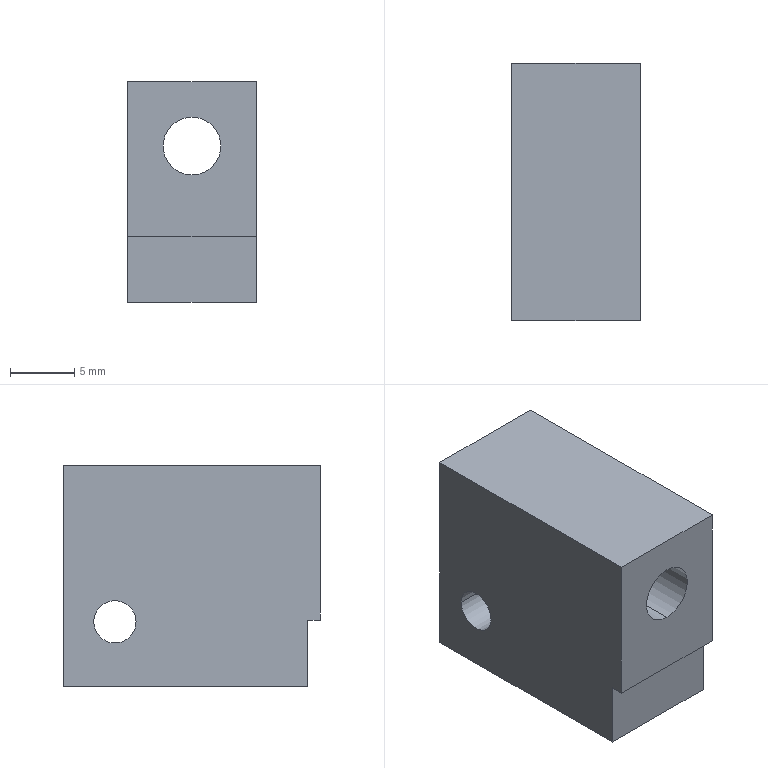Component | SolidWorks | 17268065-1 | 1 solid | 15 faces | box 10 x 20 x 17.15 mm | volume 2824 mm3 | plane 9 | cylinder 6 | commonest cylinder face diameters 3.3 x2 8 x2 4.5 x2 | material SKD-11 HRC58° Hard Chrome Plated
build123d program:
from build123d import *

# Parameters (mm, degrees)
SKETCH1_W                                       = 17.149
SKETCH1_H                                       = 10
BOSS_EXTRUDE1_DEPTH                             = 20
SKETCH2_W                                       = 5.149
SKETCH2_H                                       = 1
CUT_EXTRUDE1_DEPTH                              = 26.377
M4_HEX_SOCKET_HEAD_CAP_SCREW_CBORE1_D           = 4.5
M4_HEX_SOCKET_HEAD_CAP_SCREW_CBORE1_CBORE_D     = 8
M4_HEX_SOCKET_HEAD_CAP_SCREW_CBORE1_CBORE_DEPTH = 4.4
M4_TAPPED_HOLE1_D                               = 3.3


with BuildPart() as part:
    # Sketch1 → Boss-Extrude1 (new body)
    with BuildSketch(Plane.XY):
        with Locations((3.425, 108.5)):
            Rectangle(SKETCH1_W, SKETCH1_H)
    extrude(amount=BOSS_EXTRUDE1_DEPTH)

    # Sketch2 → Cut-Extrude1 (cut, through all)
    with BuildSketch(Plane(origin=(0, 113.5, 0), x_dir=(1, 0, 0), z_dir=(0, 1, 0))):
        with Locations((9.425, -0.5)):
            Rectangle(SKETCH2_W, SKETCH2_H)
    extrude(amount=-CUT_EXTRUDE1_DEPTH, mode=Mode.SUBTRACT)

    # M4 Hex Socket Head Cap Screw CBORE1 (through all)
    with Locations(Plane.XY.offset(20)):
        with Locations((-0.1493, 108.5)):
            CounterBoreHole(M4_HEX_SOCKET_HEAD_CAP_SCREW_CBORE1_D / 2, M4_HEX_SOCKET_HEAD_CAP_SCREW_CBORE1_CBORE_D / 2, M4_HEX_SOCKET_HEAD_CAP_SCREW_CBORE1_CBORE_DEPTH)

    # M4 Tapped Hole1 (through all)
    with Locations(Plane(origin=(0, 113.5, 0), x_dir=(1, 0, 0), z_dir=(0, 1, 0))):
        with Locations((7, -16)):
            Hole(M4_TAPPED_HOLE1_D / 2)


solid = part.part

# Placed as in the assembly
solid = solid.moved(Location((39.5, -43.579, 0.8507), (-90, 0, 90)))
STEP:
#1=COLOUR_RGB('',0.7922,0.8196,0.9333);
#2=FILL_AREA_STYLE_COLOUR('',#1);
#3=FILL_AREA_STYLE('',(#2));
#4=SURFACE_STYLE_FILL_AREA(#3);
#5=SURFACE_SIDE_STYLE('',(#4));
#6=SURFACE_STYLE_USAGE(.BOTH.,#5);
#7=PRESENTATION_STYLE_ASSIGNMENT((#6));
#8=CARTESIAN_POINT('',(-2.52,-1.151,-0.2421));
#9=VERTEX_POINT('',#8);
#10=CARTESIAN_POINT('',(-2.52,-1.021,-0.2421));
#11=VERTEX_POINT('',#10);
#12=CARTESIAN_POINT('',(-2.52,-1.086,-0.2421));
#13=DIRECTION('',(-1.,0.,0.));
#14=DIRECTION('',(0.,1.,0.));
#15=AXIS2_PLACEMENT_3D('',#12,#13,#14);
#16=CIRCLE('',#15,0.06496);
#17=EDGE_CURVE('',#9,#11,#16,.T.);
#18=ORIENTED_EDGE('',*,*,#17,.F.);
#19=CARTESIAN_POINT('',(-2.913,-1.151,-0.2421));
#20=VERTEX_POINT('',#19);
#21=CARTESIAN_POINT('',(-2.913,-1.151,-0.2421));
#22=DIRECTION('',(-1.,0.,0.));
#23=VECTOR('',#22,39.37);
#24=LINE('',#21,#23);
#25=EDGE_CURVE('',#9,#20,#24,.T.);
#26=ORIENTED_EDGE('',*,*,#25,.T.);
#27=CARTESIAN_POINT('',(-2.913,-1.021,-0.2421));
#28=VERTEX_POINT('',#27);
#29=CARTESIAN_POINT('',(-2.913,-1.086,-0.2421));
#30=DIRECTION('',(-1.,0.,0.));
#31=DIRECTION('',(0.,1.,0.));
#32=AXIS2_PLACEMENT_3D('',#29,#30,#31);
#33=CIRCLE('',#32,0.06496);
#34=EDGE_CURVE('',#20,#28,#33,.T.);
#35=ORIENTED_EDGE('',*,*,#34,.T.);
#36=CARTESIAN_POINT('',(-2.913,-1.021,-0.2421));
#37=DIRECTION('',(-1.,0.,0.));
#38=VECTOR('',#37,39.37);
#39=LINE('',#36,#38);
#40=EDGE_CURVE('',#11,#28,#39,.T.);
#41=ORIENTED_EDGE('',*,*,#40,.F.);
#42=EDGE_LOOP('',(#18,#26,#35,#41));
#43=FACE_OUTER_BOUND('',#42,.T.);
#44=CARTESIAN_POINT('',(-2.913,-1.086,-0.2421));
#45=DIRECTION('',(-1.,0.,0.));
#46=DIRECTION('',(0.,1.,0.));
#47=AXIS2_PLACEMENT_3D('',#44,#45,#46);
#48=CYLINDRICAL_SURFACE('',#47,0.06496);
#49=ADVANCED_FACE('',(#43),#48,.F.);
#50=CARTESIAN_POINT('',(-2.717,-1.102,0.1969));
#51=VERTEX_POINT('',#50);
#52=CARTESIAN_POINT('',(-2.717,-1.102,-0.1181));
#53=VERTEX_POINT('',#52);
#54=CARTESIAN_POINT('',(-2.717,-1.102,0.03937));
#55=DIRECTION('',(0.,1.,-0.));
#56=DIRECTION('',(0.,0.,-1.));
#57=AXIS2_PLACEMENT_3D('',#54,#55,#56);
#58=CIRCLE('',#57,0.1575);
#59=EDGE_CURVE('',#51,#53,#58,.T.);
#60=ORIENTED_EDGE('',*,*,#59,.F.);
#61=CARTESIAN_POINT('',(-2.717,-0.9283,0.1969));
#62=VERTEX_POINT('',#61);
#63=CARTESIAN_POINT('',(-2.717,-0.9283,0.1969));
#64=DIRECTION('',(0.,1.,-0.));
#65=VECTOR('',#64,39.37);
#66=LINE('',#63,#65);
#67=EDGE_CURVE('',#51,#62,#66,.T.);
#68=ORIENTED_EDGE('',*,*,#67,.T.);
#69=CARTESIAN_POINT('',(-2.717,-0.9283,-0.1181));
#70=VERTEX_POINT('',#69);
#71=CARTESIAN_POINT('',(-2.717,-0.9283,0.03937));
#72=DIRECTION('',(0.,1.,-0.));
#73=DIRECTION('',(0.,0.,-1.));
#74=AXIS2_PLACEMENT_3D('',#71,#72,#73);
#75=CIRCLE('',#74,0.1575);
#76=EDGE_CURVE('',#62,#70,#75,.T.);
#77=ORIENTED_EDGE('',*,*,#76,.T.);
#78=CARTESIAN_POINT('',(-2.717,-0.9283,-0.1181));
#79=DIRECTION('',(0.,1.,-0.));
#80=VECTOR('',#79,39.37);
#81=LINE('',#78,#80);
#82=EDGE_CURVE('',#53,#70,#81,.T.);
#83=ORIENTED_EDGE('',*,*,#82,.F.);
#84=EDGE_LOOP('',(#60,#68,#77,#83));
#85=FACE_OUTER_BOUND('',#84,.T.);
#86=CARTESIAN_POINT('',(-2.717,-0.9283,0.03937));
#87=DIRECTION('',(0.,1.,-0.));
#88=DIRECTION('',(0.,0.,-1.));
#89=AXIS2_PLACEMENT_3D('',#86,#87,#88);
#90=CYLINDRICAL_SURFACE('',#89,0.1575);
#91=ADVANCED_FACE('',(#85),#90,.F.);
#92=CARTESIAN_POINT('',(-2.717,-1.716,0.128));
#93=VERTEX_POINT('',#92);
#94=CARTESIAN_POINT('',(-2.717,-1.716,-0.04921));
#95=VERTEX_POINT('',#94);
#96=CARTESIAN_POINT('',(-2.717,-1.716,0.03937));
#97=DIRECTION('',(0.,1.,-0.));
#98=DIRECTION('',(0.,0.,-1.));
#99=AXIS2_PLACEMENT_3D('',#96,#97,#98);
#100=CIRCLE('',#99,0.08858);
#101=EDGE_CURVE('',#93,#95,#100,.T.);
#102=ORIENTED_EDGE('',*,*,#101,.F.);
#103=CARTESIAN_POINT('',(-2.717,-1.102,0.128));
#104=VERTEX_POINT('',#103);
#105=CARTESIAN_POINT('',(-2.717,-0.9283,0.128));
#106=DIRECTION('',(0.,1.,-0.));
#107=VECTOR('',#106,39.37);
#108=LINE('',#105,#107);
#109=EDGE_CURVE('',#93,#104,#108,.T.);
#110=ORIENTED_EDGE('',*,*,#109,.T.);
#111=CARTESIAN_POINT('',(-2.717,-1.102,-0.04921));
#112=VERTEX_POINT('',#111);
#113=CARTESIAN_POINT('',(-2.717,-1.102,0.03937));
#114=DIRECTION('',(0.,1.,-0.));
#115=DIRECTION('',(0.,0.,-1.));
#116=AXIS2_PLACEMENT_3D('',#113,#114,#115);
#117=CIRCLE('',#116,0.08858);
#118=EDGE_CURVE('',#104,#112,#117,.T.);
#119=ORIENTED_EDGE('',*,*,#118,.T.);
#120=CARTESIAN_POINT('',(-2.717,-0.9283,-0.04921));
#121=DIRECTION('',(0.,1.,-0.));
#122=VECTOR('',#121,39.37);
#123=LINE('',#120,#122);
#124=EDGE_CURVE('',#95,#112,#123,.T.);
#125=ORIENTED_EDGE('',*,*,#124,.F.);
#126=EDGE_LOOP('',(#102,#110,#119,#125));
#127=FACE_OUTER_BOUND('',#126,.T.);
#128=CARTESIAN_POINT('',(-2.717,-0.9283,0.03937));
#129=DIRECTION('',(0.,1.,-0.));
#130=DIRECTION('',(0.,0.,-1.));
#131=AXIS2_PLACEMENT_3D('',#128,#129,#130);
#132=CYLINDRICAL_SURFACE('',#131,0.08858);
#133=ADVANCED_FACE('',(#127),#132,.F.);
#134=CARTESIAN_POINT('',(-2.913,-1.716,0.2362));
#135=VERTEX_POINT('',#134);
#136=CARTESIAN_POINT('',(-2.52,-1.716,0.2362));
#137=VERTEX_POINT('',#136);
#138=CARTESIAN_POINT('',(-2.913,-1.716,0.2362));
#139=DIRECTION('',(1.,-0.,-0.));
#140=VECTOR('',#139,39.37);
#141=LINE('',#138,#140);
#142=EDGE_CURVE('',#135,#137,#141,.T.);
#143=ORIENTED_EDGE('',*,*,#142,.T.);
#144=CARTESIAN_POINT('',(-2.52,-0.9283,0.2362));
#145=VERTEX_POINT('',#144);
#146=CARTESIAN_POINT('',(-2.52,-0.9283,0.2362));
#147=DIRECTION('',(0.,-1.,0.));
#148=VECTOR('',#147,39.37);
#149=LINE('',#146,#148);
#150=EDGE_CURVE('',#145,#137,#149,.T.);
#151=ORIENTED_EDGE('',*,*,#150,.F.);
#152=CARTESIAN_POINT('',(-2.913,-0.9283,0.2362));
#153=VERTEX_POINT('',#152);
#154=CARTESIAN_POINT('',(-2.913,-0.9283,0.2362));
#155=DIRECTION('',(1.,-0.,-0.));
#156=VECTOR('',#155,39.37);
#157=LINE('',#154,#156);
#158=EDGE_CURVE('',#153,#145,#157,.T.);
#159=ORIENTED_EDGE('',*,*,#158,.F.);
#160=CARTESIAN_POINT('',(-2.913,-0.9283,0.2362));
#161=DIRECTION('',(0.,-1.,0.));
#162=VECTOR('',#161,39.37);
#163=LINE('',#160,#162);
#164=EDGE_CURVE('',#153,#135,#163,.T.);
#165=ORIENTED_EDGE('',*,*,#164,.T.);
#166=EDGE_LOOP('',(#143,#151,#159,#165));
#167=FACE_OUTER_BOUND('',#166,.T.);
#168=CARTESIAN_POINT('',(-2.913,-0.9283,0.2362));
#169=DIRECTION('',(-0.,-0.,-1.));
#170=DIRECTION('',(-1.,0.,0.));
#171=AXIS2_PLACEMENT_3D('',#168,#169,#170);
#172=PLANE('',#171);
#173=ADVANCED_FACE('',(#167),#172,.F.);
#174=CARTESIAN_POINT('',(-2.52,-1.086,-0.2421));
#175=DIRECTION('',(-1.,0.,0.));
#176=DIRECTION('',(0.,1.,0.));
#177=AXIS2_PLACEMENT_3D('',#174,#175,#176);
#178=CIRCLE('',#177,0.06496);
#179=EDGE_CURVE('',#11,#9,#178,.T.);
#180=ORIENTED_EDGE('',*,*,#179,.T.);
#181=ORIENTED_EDGE('',*,*,#17,.T.);
#182=EDGE_LOOP('',(#180,#181));
#183=FACE_BOUND('',#182,.T.);
#184=CARTESIAN_POINT('',(-2.52,-1.716,-0.2362));
#185=VERTEX_POINT('',#184);
#186=CARTESIAN_POINT('',(-2.52,-1.716,0.2362));
#187=DIRECTION('',(0.,-0.,-1.));
#188=VECTOR('',#187,39.37);
#189=LINE('',#186,#188);
#190=EDGE_CURVE('',#137,#185,#189,.T.);
#191=ORIENTED_EDGE('',*,*,#190,.T.);
#192=CARTESIAN_POINT('',(-2.52,-1.676,-0.2362));
#193=VERTEX_POINT('',#192);
#194=CARTESIAN_POINT('',(-2.52,-1.716,-0.2362));
#195=DIRECTION('',(0.,1.,-0.));
#196=VECTOR('',#195,39.37);
#197=LINE('',#194,#196);
#198=EDGE_CURVE('',#185,#193,#197,.T.);
#199=ORIENTED_EDGE('',*,*,#198,.T.);
#200=CARTESIAN_POINT('',(-2.52,-1.676,-0.4389));
#201=VERTEX_POINT('',#200);
#202=CARTESIAN_POINT('',(-2.52,-1.676,-0.2362));
#203=DIRECTION('',(0.,-0.,-1.));
#204=VECTOR('',#203,39.37);
#205=LINE('',#202,#204);
#206=EDGE_CURVE('',#193,#201,#205,.T.);
#207=ORIENTED_EDGE('',*,*,#206,.T.);
#208=CARTESIAN_POINT('',(-2.52,-0.9283,-0.4389));
#209=VERTEX_POINT('',#208);
#210=CARTESIAN_POINT('',(-2.52,-0.9283,-0.4389));
#211=DIRECTION('',(0.,-1.,0.));
#212=VECTOR('',#211,39.37);
#213=LINE('',#210,#212);
#214=EDGE_CURVE('',#209,#201,#213,.T.);
#215=ORIENTED_EDGE('',*,*,#214,.F.);
#216=CARTESIAN_POINT('',(-2.52,-0.9283,0.2362));
#217=DIRECTION('',(0.,-0.,-1.));
#218=VECTOR('',#217,39.37);
#219=LINE('',#216,#218);
#220=EDGE_CURVE('',#145,#209,#219,.T.);
#221=ORIENTED_EDGE('',*,*,#220,.F.);
#222=ORIENTED_EDGE('',*,*,#150,.T.);
#223=EDGE_LOOP('',(#191,#199,#207,#215,#221,#222));
#224=FACE_OUTER_BOUND('',#223,.T.);
#225=CARTESIAN_POINT('',(-2.52,-0.9283,0.2362));
#226=DIRECTION('',(-1.,0.,0.));
#227=DIRECTION('',(0.,1.,-0.));
#228=AXIS2_PLACEMENT_3D('',#225,#226,#227);
#229=PLANE('',#228);
#230=ADVANCED_FACE('',(#183,#224),#229,.F.);
#231=ORIENTED_EDGE('',*,*,#214,.T.);
#232=CARTESIAN_POINT('',(-2.913,-1.676,-0.4389));
#233=VERTEX_POINT('',#232);
#234=CARTESIAN_POINT('',(-2.52,-1.676,-0.4389));
#235=DIRECTION('',(-1.,0.,0.));
#236=VECTOR('',#235,39.37);
#237=LINE('',#234,#236);
#238=EDGE_CURVE('',#201,#233,#237,.T.);
#239=ORIENTED_EDGE('',*,*,#238,.T.);
#240=CARTESIAN_POINT('',(-2.913,-0.9283,-0.4389));
#241=VERTEX_POINT('',#240);
#242=CARTESIAN_POINT('',(-2.913,-0.9283,-0.4389));
#243=DIRECTION('',(0.,-1.,0.));
#244=VECTOR('',#243,39.37);
#245=LINE('',#242,#244);
#246=EDGE_CURVE('',#241,#233,#245,.T.);
#247=ORIENTED_EDGE('',*,*,#246,.F.);
#248=CARTESIAN_POINT('',(-2.913,-0.9283,-0.4389));
#249=DIRECTION('',(-1.,0.,0.));
#250=VECTOR('',#249,39.37);
#251=LINE('',#248,#250);
#252=EDGE_CURVE('',#209,#241,#251,.T.);
#253=ORIENTED_EDGE('',*,*,#252,.F.);
#254=EDGE_LOOP('',(#231,#239,#247,#253));
#255=FACE_OUTER_BOUND('',#254,.T.);
#256=CARTESIAN_POINT('',(-2.913,-0.9283,-0.4389));
#257=DIRECTION('',(0.,0.,1.));
#258=DIRECTION('',(0.,1.,-0.));
#259=AXIS2_PLACEMENT_3D('',#256,#257,#258);
#260=PLANE('',#259);
#261=ADVANCED_FACE('',(#255),#260,.F.);
#262=CARTESIAN_POINT('',(-2.913,-1.086,-0.2421));
#263=DIRECTION('',(-1.,0.,0.));
#264=DIRECTION('',(0.,1.,0.));
#265=AXIS2_PLACEMENT_3D('',#262,#263,#264);
#266=CIRCLE('',#265,0.06496);
#267=EDGE_CURVE('',#28,#20,#266,.T.);
#268=ORIENTED_EDGE('',*,*,#267,.F.);
#269=ORIENTED_EDGE('',*,*,#34,.F.);
#270=EDGE_LOOP('',(#268,#269));
#271=FACE_BOUND('',#270,.T.);
#272=CARTESIAN_POINT('',(-2.913,-1.676,-0.2362));
#273=VERTEX_POINT('',#272);
#274=CARTESIAN_POINT('',(-2.913,-1.676,-0.2362));
#275=DIRECTION('',(0.,-0.,-1.));
#276=VECTOR('',#275,39.37);
#277=LINE('',#274,#276);
#278=EDGE_CURVE('',#273,#233,#277,.T.);
#279=ORIENTED_EDGE('',*,*,#278,.F.);
#280=CARTESIAN_POINT('',(-2.913,-1.716,-0.2362));
#281=VERTEX_POINT('',#280);
#282=CARTESIAN_POINT('',(-2.913,-1.716,-0.2362));
#283=DIRECTION('',(0.,1.,-0.));
#284=VECTOR('',#283,39.37);
#285=LINE('',#282,#284);
#286=EDGE_CURVE('',#281,#273,#285,.T.);
#287=ORIENTED_EDGE('',*,*,#286,.F.);
#288=CARTESIAN_POINT('',(-2.913,-1.716,0.2362));
#289=DIRECTION('',(0.,0.,1.));
#290=VECTOR('',#289,39.37);
#291=LINE('',#288,#290);
#292=EDGE_CURVE('',#281,#135,#291,.T.);
#293=ORIENTED_EDGE('',*,*,#292,.T.);
#294=ORIENTED_EDGE('',*,*,#164,.F.);
#295=CARTESIAN_POINT('',(-2.913,-0.9283,0.2362));
#296=DIRECTION('',(0.,0.,1.));
#297=VECTOR('',#296,39.37);
#298=LINE('',#295,#297);
#299=EDGE_CURVE('',#241,#153,#298,.T.);
#300=ORIENTED_EDGE('',*,*,#299,.F.);
#301=ORIENTED_EDGE('',*,*,#246,.T.);
#302=EDGE_LOOP('',(#279,#287,#293,#294,#300,#301));
#303=FACE_OUTER_BOUND('',#302,.T.);
#304=CARTESIAN_POINT('',(-2.913,-0.9283,0.2362));
#305=DIRECTION('',(1.,0.,0.));
#306=DIRECTION('',(0.,-1.,0.));
#307=AXIS2_PLACEMENT_3D('',#304,#305,#306);
#308=PLANE('',#307);
#309=ADVANCED_FACE('',(#271,#303),#308,.F.);
#310=CARTESIAN_POINT('',(-2.717,-0.9283,0.03937));
#311=DIRECTION('',(0.,1.,-0.));
#312=DIRECTION('',(0.,0.,-1.));
#313=AXIS2_PLACEMENT_3D('',#310,#311,#312);
#314=CIRCLE('',#313,0.1575);
#315=EDGE_CURVE('',#70,#62,#314,.T.);
#316=ORIENTED_EDGE('',*,*,#315,.F.);
#317=ORIENTED_EDGE('',*,*,#76,.F.);
#318=EDGE_LOOP('',(#316,#317));
#319=FACE_BOUND('',#318,.T.);
#320=ORIENTED_EDGE('',*,*,#158,.T.);
#321=ORIENTED_EDGE('',*,*,#220,.T.);
#322=ORIENTED_EDGE('',*,*,#252,.T.);
#323=ORIENTED_EDGE('',*,*,#299,.T.);
#324=EDGE_LOOP('',(#320,#321,#322,#323));
#325=FACE_OUTER_BOUND('',#324,.T.);
#326=CARTESIAN_POINT('',(1.555,-0.9283,0.03349));
#327=DIRECTION('',(0.,1.,-0.));
#328=DIRECTION('',(0.,-0.,-1.));
#329=AXIS2_PLACEMENT_3D('',#326,#327,#328);
#330=PLANE('',#329);
#331=ADVANCED_FACE('',(#319,#325),#330,.T.);
#332=CARTESIAN_POINT('',(-2.717,-1.716,0.03937));
#333=DIRECTION('',(0.,1.,-0.));
#334=DIRECTION('',(0.,0.,-1.));
#335=AXIS2_PLACEMENT_3D('',#332,#333,#334);
#336=CIRCLE('',#335,0.08858);
#337=EDGE_CURVE('',#95,#93,#336,.T.);
#338=ORIENTED_EDGE('',*,*,#337,.T.);
#339=ORIENTED_EDGE('',*,*,#101,.T.);
#340=EDGE_LOOP('',(#338,#339));
#341=FACE_BOUND('',#340,.T.);
#342=ORIENTED_EDGE('',*,*,#292,.F.);
#343=CARTESIAN_POINT('',(-2.52,-1.716,-0.2362));
#344=DIRECTION('',(-1.,0.,0.));
#345=VECTOR('',#344,39.37);
#346=LINE('',#343,#345);
#347=EDGE_CURVE('',#185,#281,#346,.T.);
#348=ORIENTED_EDGE('',*,*,#347,.F.);
#349=ORIENTED_EDGE('',*,*,#190,.F.);
#350=ORIENTED_EDGE('',*,*,#142,.F.);
#351=EDGE_LOOP('',(#342,#348,#349,#350));
#352=FACE_OUTER_BOUND('',#351,.T.);
#353=CARTESIAN_POINT('',(1.555,-1.716,0.03349));
#354=DIRECTION('',(0.,1.,-0.));
#355=DIRECTION('',(0.,-0.,-1.));
#356=AXIS2_PLACEMENT_3D('',#353,#354,#355);
#357=PLANE('',#356);
#358=ADVANCED_FACE('',(#341,#352),#357,.F.);
#359=ORIENTED_EDGE('',*,*,#286,.T.);
#360=CARTESIAN_POINT('',(-2.52,-1.676,-0.2362));
#361=DIRECTION('',(-1.,0.,0.));
#362=VECTOR('',#361,39.37);
#363=LINE('',#360,#362);
#364=EDGE_CURVE('',#193,#273,#363,.T.);
#365=ORIENTED_EDGE('',*,*,#364,.F.);
#366=ORIENTED_EDGE('',*,*,#198,.F.);
#367=ORIENTED_EDGE('',*,*,#347,.T.);
#368=EDGE_LOOP('',(#359,#365,#366,#367));
#369=FACE_OUTER_BOUND('',#368,.T.);
#370=CARTESIAN_POINT('',(-2.52,-1.716,-0.2362));
#371=DIRECTION('',(0.,0.,1.));
#372=DIRECTION('',(0.,1.,-0.));
#373=AXIS2_PLACEMENT_3D('',#370,#371,#372);
#374=PLANE('',#373);
#375=ADVANCED_FACE('',(#369),#374,.F.);
#376=ORIENTED_EDGE('',*,*,#278,.T.);
#377=ORIENTED_EDGE('',*,*,#238,.F.);
#378=ORIENTED_EDGE('',*,*,#206,.F.);
#379=ORIENTED_EDGE('',*,*,#364,.T.);
#380=EDGE_LOOP('',(#376,#377,#378,#379));
#381=FACE_OUTER_BOUND('',#380,.T.);
#382=CARTESIAN_POINT('',(-2.52,-1.676,-0.2362));
#383=DIRECTION('',(0.,1.,-0.));
#384=DIRECTION('',(0.,-0.,-1.));
#385=AXIS2_PLACEMENT_3D('',#382,#383,#384);
#386=PLANE('',#385);
#387=ADVANCED_FACE('',(#381),#386,.F.);
#388=ORIENTED_EDGE('',*,*,#109,.F.);
#389=ORIENTED_EDGE('',*,*,#337,.F.);
#390=ORIENTED_EDGE('',*,*,#124,.T.);
#391=CARTESIAN_POINT('',(-2.717,-1.102,0.03937));
#392=DIRECTION('',(0.,1.,-0.));
#393=DIRECTION('',(0.,0.,-1.));
#394=AXIS2_PLACEMENT_3D('',#391,#392,#393);
#395=CIRCLE('',#394,0.08858);
#396=EDGE_CURVE('',#112,#104,#395,.T.);
#397=ORIENTED_EDGE('',*,*,#396,.T.);
#398=EDGE_LOOP('',(#388,#389,#390,#397));
#399=FACE_OUTER_BOUND('',#398,.T.);
#400=CARTESIAN_POINT('',(-2.717,-0.9283,0.03937));
#401=DIRECTION('',(0.,1.,-0.));
#402=DIRECTION('',(0.,0.,-1.));
#403=AXIS2_PLACEMENT_3D('',#400,#401,#402);
#404=CYLINDRICAL_SURFACE('',#403,0.08858);
#405=ADVANCED_FACE('',(#399),#404,.F.);
#406=ORIENTED_EDGE('',*,*,#396,.F.);
#407=ORIENTED_EDGE('',*,*,#118,.F.);
#408=EDGE_LOOP('',(#406,#407));
#409=FACE_BOUND('',#408,.T.);
#410=CARTESIAN_POINT('',(-2.717,-1.102,0.03937));
#411=DIRECTION('',(0.,1.,-0.));
#412=DIRECTION('',(0.,0.,-1.));
#413=AXIS2_PLACEMENT_3D('',#410,#411,#412);
#414=CIRCLE('',#413,0.1575);
#415=EDGE_CURVE('',#53,#51,#414,.T.);
#416=ORIENTED_EDGE('',*,*,#415,.T.);
#417=ORIENTED_EDGE('',*,*,#59,.T.);
#418=EDGE_LOOP('',(#416,#417));
#419=FACE_OUTER_BOUND('',#418,.T.);
#420=CARTESIAN_POINT('',(-2.717,-1.102,-0.04921));
#421=DIRECTION('',(0.,-1.,0.));
#422=DIRECTION('',(0.,0.,1.));
#423=AXIS2_PLACEMENT_3D('',#420,#421,#422);
#424=PLANE('',#423);
#425=ADVANCED_FACE('',(#409,#419),#424,.F.);
#426=ORIENTED_EDGE('',*,*,#67,.F.);
#427=ORIENTED_EDGE('',*,*,#415,.F.);
#428=ORIENTED_EDGE('',*,*,#82,.T.);
#429=ORIENTED_EDGE('',*,*,#315,.T.);
#430=EDGE_LOOP('',(#426,#427,#428,#429));
#431=FACE_OUTER_BOUND('',#430,.T.);
#432=CARTESIAN_POINT('',(-2.717,-0.9283,0.03937));
#433=DIRECTION('',(0.,1.,-0.));
#434=DIRECTION('',(0.,0.,-1.));
#435=AXIS2_PLACEMENT_3D('',#432,#433,#434);
#436=CYLINDRICAL_SURFACE('',#435,0.1575);
#437=ADVANCED_FACE('',(#431),#436,.F.);
#438=ORIENTED_EDGE('',*,*,#25,.F.);
#439=ORIENTED_EDGE('',*,*,#179,.F.);
#440=ORIENTED_EDGE('',*,*,#40,.T.);
#441=ORIENTED_EDGE('',*,*,#267,.T.);
#442=EDGE_LOOP('',(#438,#439,#440,#441));
#443=FACE_OUTER_BOUND('',#442,.T.);
#444=CARTESIAN_POINT('',(-2.913,-1.086,-0.2421));
#445=DIRECTION('',(-1.,0.,0.));
#446=DIRECTION('',(0.,1.,0.));
#447=AXIS2_PLACEMENT_3D('',#444,#445,#446);
#448=CYLINDRICAL_SURFACE('',#447,0.06496);
#449=ADVANCED_FACE('',(#443),#448,.F.);
#450=CLOSED_SHELL('',(#49,#91,#133,#173,#230,#261,#309,#331,#358,#375,#387,#405,#425,#437,#449));
#451=MANIFOLD_SOLID_BREP('',#450);
#452=STYLED_ITEM('',(#7),#451);
#453=PRESENTATION_LAYER_ASSIGNMENT('','',(#452));
#454=(LENGTH_UNIT()NAMED_UNIT(*)SI_UNIT($,.METRE.));
#455=LENGTH_MEASURE_WITH_UNIT(LENGTH_MEASURE(0.0254),#454);
#456=DIMENSIONAL_EXPONENTS(1.,0.,0.,0.,0.,0.,0.);
#457=(CONVERSION_BASED_UNIT('',#455)LENGTH_UNIT()NAMED_UNIT(#456));
#458=UNCERTAINTY_MEASURE_WITH_UNIT(LENGTH_MEASURE(0.00001),#457,'','');
#459=(NAMED_UNIT(*)PLANE_ANGLE_UNIT()SI_UNIT($,.RADIAN.));
#460=(NAMED_UNIT(*)SI_UNIT($,.STERADIAN.)SOLID_ANGLE_UNIT());
#461=(GEOMETRIC_REPRESENTATION_CONTEXT(3)GLOBAL_UNCERTAINTY_ASSIGNED_CONTEXT((#458))GLOBAL_UNIT_ASSIGNED_CONTEXT((#457,#459,#460))REPRESENTATION_CONTEXT('',''));
#462=MECHANICAL_DESIGN_GEOMETRIC_PRESENTATION_REPRESENTATION('',(#452),#461);
#463=CARTESIAN_POINT('',(0.,0.,0.));
#464=DIRECTION('',(0.,0.,1.));
#465=DIRECTION('',(1.,0.,0.));
#466=AXIS2_PLACEMENT_3D('',#463,#464,#465);
#467=(LENGTH_UNIT()NAMED_UNIT(*)SI_UNIT($,.METRE.));
#468=LENGTH_MEASURE_WITH_UNIT(LENGTH_MEASURE(0.0254),#467);
#469=DIMENSIONAL_EXPONENTS(1.,0.,0.,0.,0.,0.,0.);
#470=(CONVERSION_BASED_UNIT('',#468)LENGTH_UNIT()NAMED_UNIT(#469));
#471=UNCERTAINTY_MEASURE_WITH_UNIT(LENGTH_MEASURE(0.00001),#470,'','');
#472=(NAMED_UNIT(*)PLANE_ANGLE_UNIT()SI_UNIT($,.RADIAN.));
#473=(NAMED_UNIT(*)SI_UNIT($,.STERADIAN.)SOLID_ANGLE_UNIT());
#474=(GEOMETRIC_REPRESENTATION_CONTEXT(3)GLOBAL_UNCERTAINTY_ASSIGNED_CONTEXT((#471))GLOBAL_UNIT_ASSIGNED_CONTEXT((#470,#472,#473))REPRESENTATION_CONTEXT('',''));
#475=ADVANCED_BREP_SHAPE_REPRESENTATION('',(#451,#466),#474);